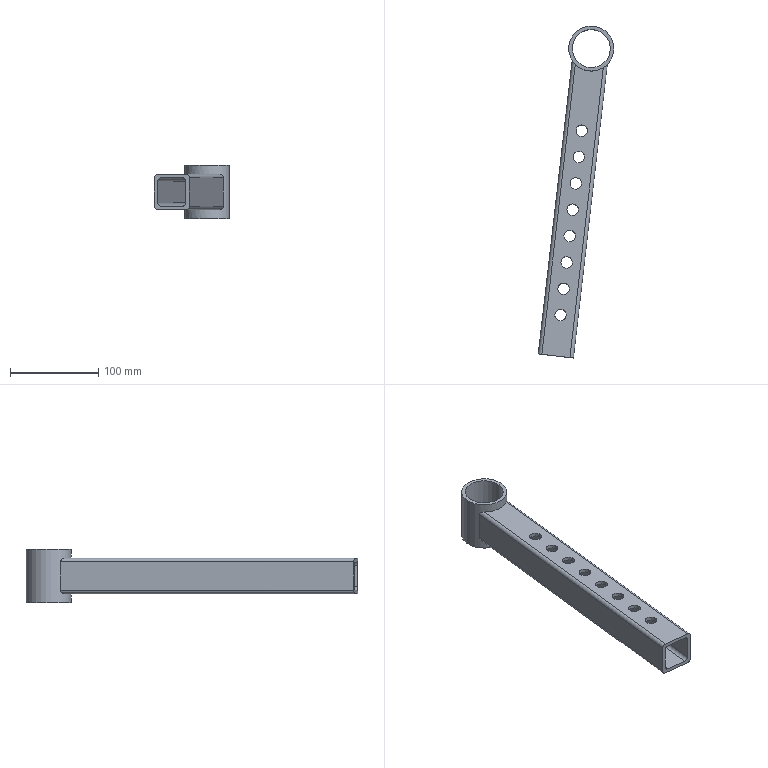Component | NX | ADJ_INNER_BRKT | 1 solid | 38 faces | volume 216668 mm3 | cylinder 27 | plane 11 | commonest cylinder face diameters 13 x16 8 x8 51 x2 43 x1